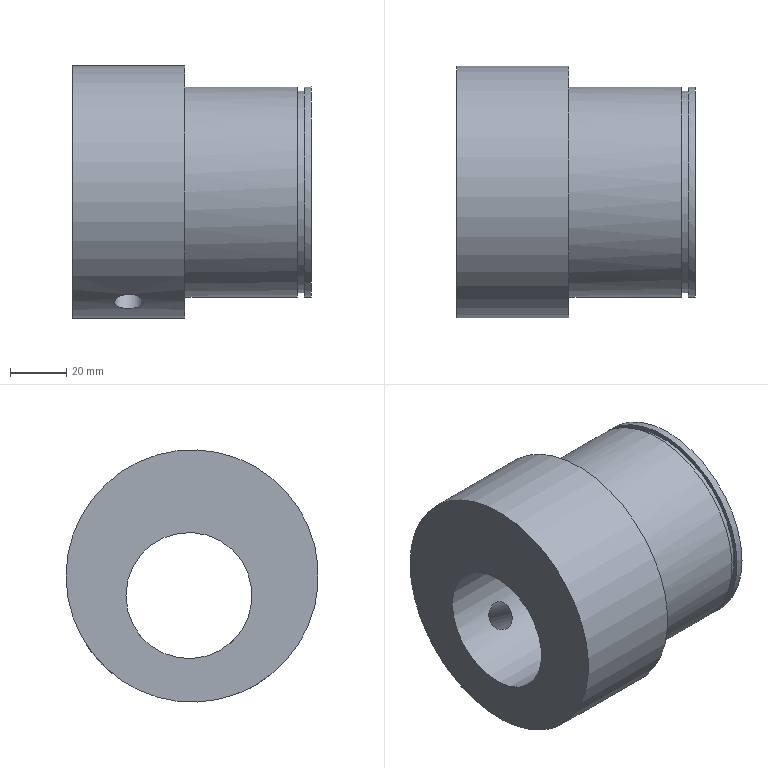Component | NX | LIMIT_SHAFT_SLEEVE_1 | 1 solid | 12 faces | volume 314395 mm3 | cylinder 7 | plane 5 | commonest cylinder face diameters 75 x2 10.2 x2 90 x1 45 x1 72 x1